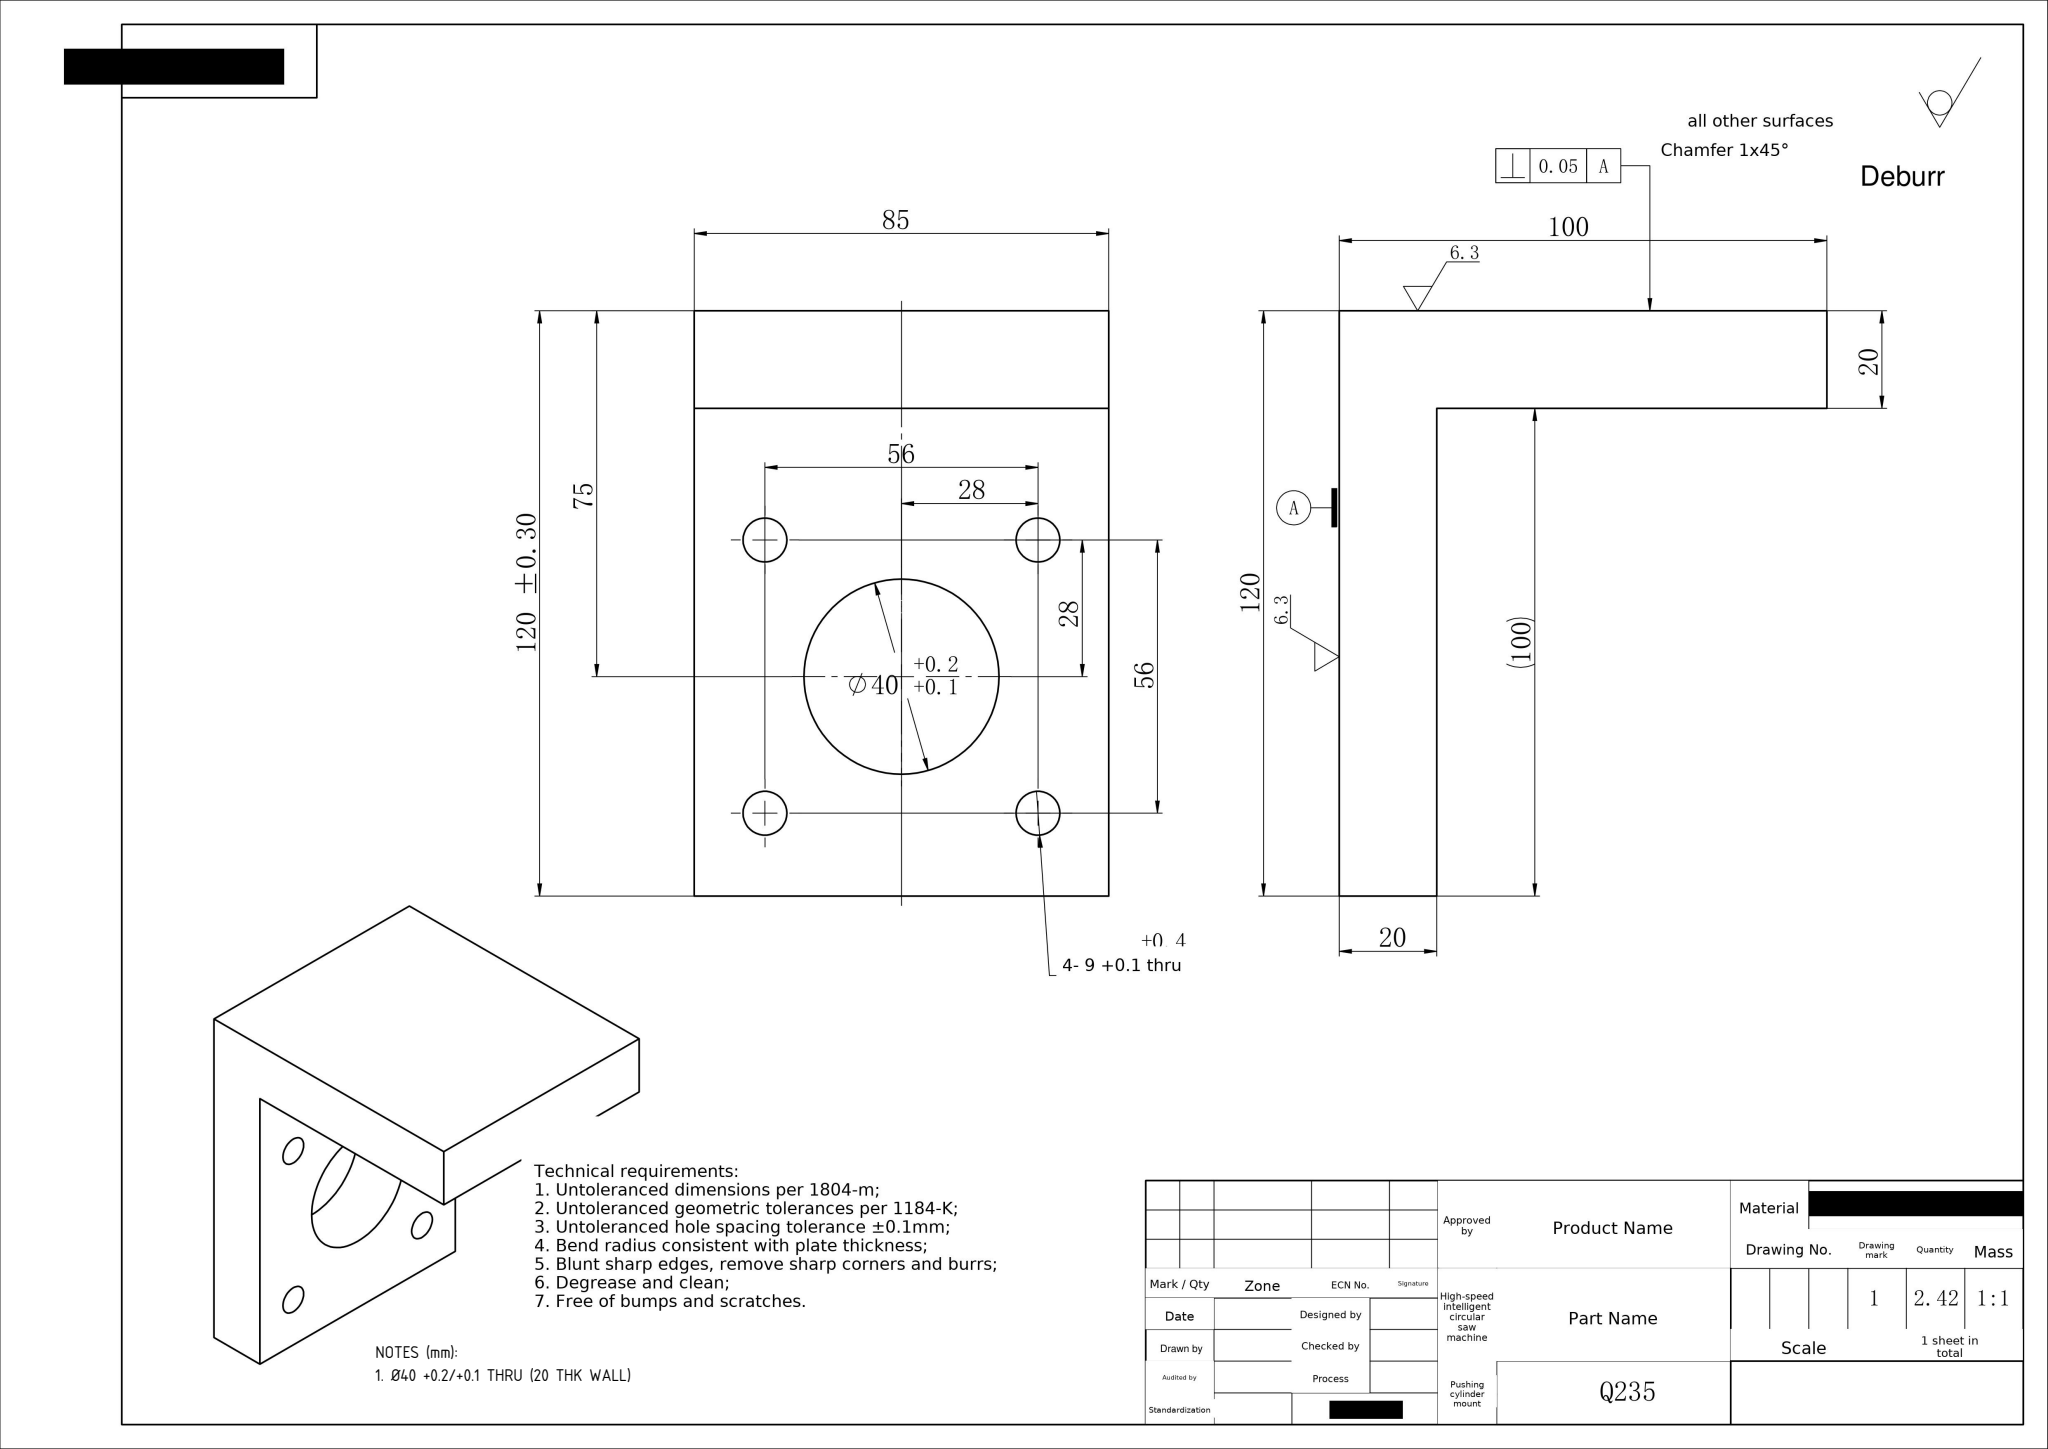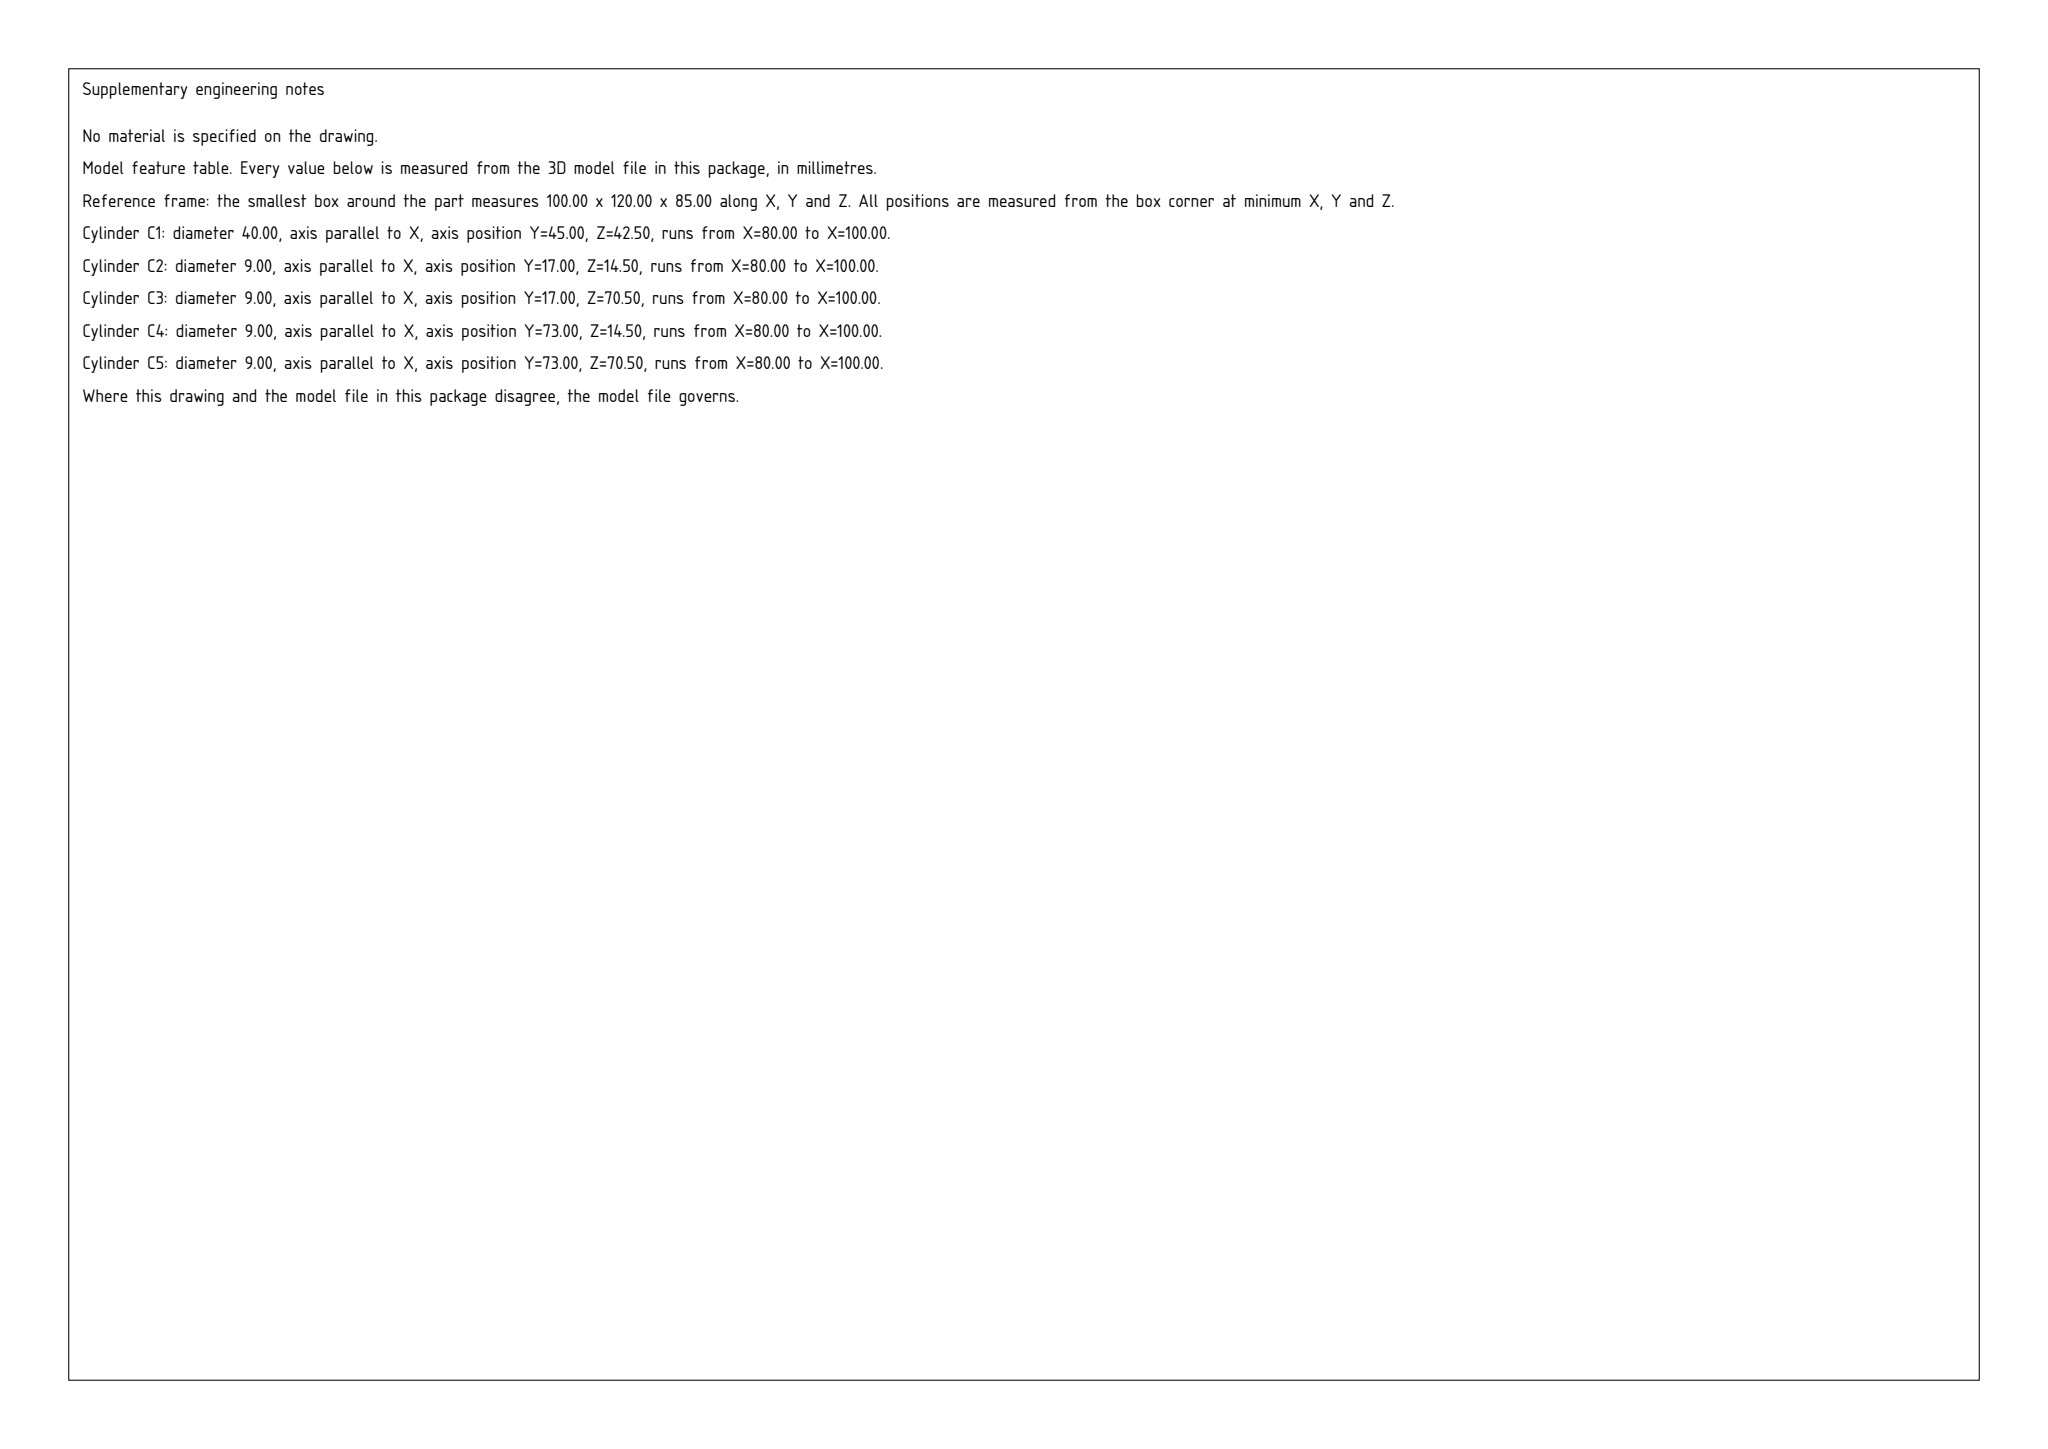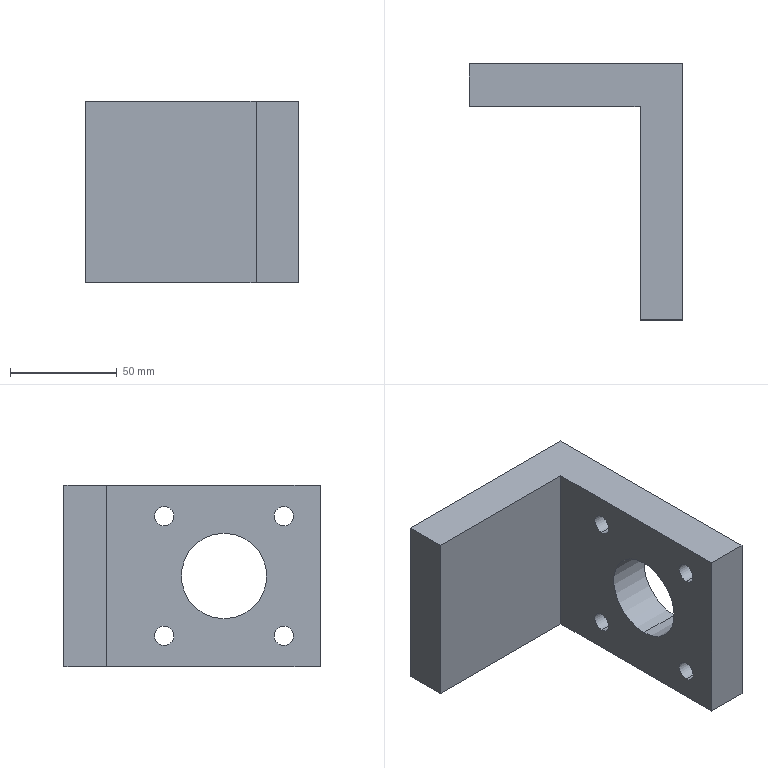Part | SolidWorks | mm | 1 solid | 18 faces | box 100 x 120 x 85 mm | volume 309778 mm3 | cylinder 10 | plane 8 | commonest cylinder face diameters 9 x8 40 x2
Drawing notes:
Ø40 +0.2/+0.1 THRU (20 THK WALL) | from the solid: 40 dia cyl, axis x, length 20.0 = wall thk (x-planes 80.0 to 100.0)
build123d program:
from build123d import *

# Parameters (mm, degrees)
BOSS_EXTRUDE1_DEPTH = 85
SKETCH2_R           = 20
SKETCH2_R_2         = 4.5
CUT_EXTRUDE1_DEPTH  = 178.834


with BuildPart() as part:
    # Sketch1 → Boss-Extrude1 (new body)
    with BuildSketch(Plane.XY):
        Polygon((0, 0), (0, 120), (-100, 120), (-100, 100), (-20, 100), (-20, 0), align=None)
    extrude(amount=BOSS_EXTRUDE1_DEPTH)

    # Sketch2 → Cut-Extrude1 (cut, through all)
    with BuildSketch(Plane(origin=(0, 0, 0), x_dir=(0, 0, -1), z_dir=(1, 0, 0))):
        with Locations((-42.5, 45)):
            Circle(SKETCH2_R)
        with Locations((-70.5, 73)):
            Circle(SKETCH2_R_2)
        with Locations((-14.5, 73)):
            Circle(SKETCH2_R_2)
        with Locations((-14.5, 17)):
            Circle(SKETCH2_R_2)
        with Locations((-70.5, 17)):
            Circle(SKETCH2_R_2)
    extrude(amount=-CUT_EXTRUDE1_DEPTH, mode=Mode.SUBTRACT)


solid = part.part
STEP:
#1=CARTESIAN_POINT('',(-20.,17.,75.));
#2=VERTEX_POINT('',#1);
#3=CARTESIAN_POINT('',(-20.,17.,66.));
#4=VERTEX_POINT('',#3);
#5=CARTESIAN_POINT('',(-20.,17.,70.5));
#6=DIRECTION('',(1.,0.,0.));
#7=DIRECTION('',(0.,0.,-1.));
#8=AXIS2_PLACEMENT_3D('',#5,#6,#7);
#9=CIRCLE('',#8,4.5);
#10=EDGE_CURVE('',#2,#4,#9,.T.);
#11=ORIENTED_EDGE('',*,*,#10,.F.);
#12=CARTESIAN_POINT('',(0.,17.,75.));
#13=VERTEX_POINT('',#12);
#14=CARTESIAN_POINT('',(-100.,17.,75.));
#15=DIRECTION('',(1.,0.,0.));
#16=VECTOR('',#15,1000.);
#17=LINE('',#14,#16);
#18=EDGE_CURVE('',#2,#13,#17,.T.);
#19=ORIENTED_EDGE('',*,*,#18,.T.);
#20=CARTESIAN_POINT('',(0.,17.,66.));
#21=VERTEX_POINT('',#20);
#22=CARTESIAN_POINT('',(0.,17.,70.5));
#23=DIRECTION('',(1.,0.,0.));
#24=DIRECTION('',(0.,0.,1.));
#25=AXIS2_PLACEMENT_3D('',#22,#23,#24);
#26=CIRCLE('',#25,4.5);
#27=EDGE_CURVE('',#13,#21,#26,.T.);
#28=ORIENTED_EDGE('',*,*,#27,.T.);
#29=CARTESIAN_POINT('',(-100.,17.,66.));
#30=DIRECTION('',(1.,0.,0.));
#31=VECTOR('',#30,1000.);
#32=LINE('',#29,#31);
#33=EDGE_CURVE('',#4,#21,#32,.T.);
#34=ORIENTED_EDGE('',*,*,#33,.F.);
#35=EDGE_LOOP('',(#11,#19,#28,#34));
#36=FACE_OUTER_BOUND('',#35,.T.);
#37=CARTESIAN_POINT('',(-100.,17.,70.5));
#38=DIRECTION('',(1.,0.,0.));
#39=DIRECTION('',(0.,0.,-1.));
#40=AXIS2_PLACEMENT_3D('',#37,#38,#39);
#41=CYLINDRICAL_SURFACE('',#40,4.5);
#42=ADVANCED_FACE('',(#36),#41,.F.);
#43=CARTESIAN_POINT('',(-20.,17.,19.));
#44=VERTEX_POINT('',#43);
#45=CARTESIAN_POINT('',(-20.,17.,10.));
#46=VERTEX_POINT('',#45);
#47=CARTESIAN_POINT('',(-20.,17.,14.5));
#48=DIRECTION('',(1.,0.,0.));
#49=DIRECTION('',(0.,0.,-1.));
#50=AXIS2_PLACEMENT_3D('',#47,#48,#49);
#51=CIRCLE('',#50,4.5);
#52=EDGE_CURVE('',#44,#46,#51,.T.);
#53=ORIENTED_EDGE('',*,*,#52,.F.);
#54=CARTESIAN_POINT('',(0.,17.,19.));
#55=VERTEX_POINT('',#54);
#56=CARTESIAN_POINT('',(-100.,17.,19.));
#57=DIRECTION('',(1.,0.,0.));
#58=VECTOR('',#57,1000.);
#59=LINE('',#56,#58);
#60=EDGE_CURVE('',#44,#55,#59,.T.);
#61=ORIENTED_EDGE('',*,*,#60,.T.);
#62=CARTESIAN_POINT('',(0.,17.,10.));
#63=VERTEX_POINT('',#62);
#64=CARTESIAN_POINT('',(0.,17.,14.5));
#65=DIRECTION('',(1.,0.,0.));
#66=DIRECTION('',(0.,0.,-1.));
#67=AXIS2_PLACEMENT_3D('',#64,#65,#66);
#68=CIRCLE('',#67,4.5);
#69=EDGE_CURVE('',#55,#63,#68,.T.);
#70=ORIENTED_EDGE('',*,*,#69,.T.);
#71=CARTESIAN_POINT('',(-100.,17.,10.));
#72=DIRECTION('',(1.,0.,0.));
#73=VECTOR('',#72,1000.);
#74=LINE('',#71,#73);
#75=EDGE_CURVE('',#46,#63,#74,.T.);
#76=ORIENTED_EDGE('',*,*,#75,.F.);
#77=EDGE_LOOP('',(#53,#61,#70,#76));
#78=FACE_OUTER_BOUND('',#77,.T.);
#79=CARTESIAN_POINT('',(-100.,17.,14.5));
#80=DIRECTION('',(1.,0.,0.));
#81=DIRECTION('',(0.,0.,-1.));
#82=AXIS2_PLACEMENT_3D('',#79,#80,#81);
#83=CYLINDRICAL_SURFACE('',#82,4.5);
#84=ADVANCED_FACE('',(#78),#83,.F.);
#85=CARTESIAN_POINT('',(-20.,73.,19.));
#86=VERTEX_POINT('',#85);
#87=CARTESIAN_POINT('',(-20.,73.,10.));
#88=VERTEX_POINT('',#87);
#89=CARTESIAN_POINT('',(-20.,73.,14.5));
#90=DIRECTION('',(1.,0.,0.));
#91=DIRECTION('',(0.,0.,-1.));
#92=AXIS2_PLACEMENT_3D('',#89,#90,#91);
#93=CIRCLE('',#92,4.5);
#94=EDGE_CURVE('',#86,#88,#93,.T.);
#95=ORIENTED_EDGE('',*,*,#94,.F.);
#96=CARTESIAN_POINT('',(0.,73.,19.));
#97=VERTEX_POINT('',#96);
#98=CARTESIAN_POINT('',(-100.,73.,19.));
#99=DIRECTION('',(1.,0.,0.));
#100=VECTOR('',#99,1000.);
#101=LINE('',#98,#100);
#102=EDGE_CURVE('',#86,#97,#101,.T.);
#103=ORIENTED_EDGE('',*,*,#102,.T.);
#104=CARTESIAN_POINT('',(0.,73.,10.));
#105=VERTEX_POINT('',#104);
#106=CARTESIAN_POINT('',(0.,73.,14.5));
#107=DIRECTION('',(1.,0.,0.));
#108=DIRECTION('',(0.,0.,1.));
#109=AXIS2_PLACEMENT_3D('',#106,#107,#108);
#110=CIRCLE('',#109,4.5);
#111=EDGE_CURVE('',#97,#105,#110,.T.);
#112=ORIENTED_EDGE('',*,*,#111,.T.);
#113=CARTESIAN_POINT('',(-100.,73.,10.));
#114=DIRECTION('',(1.,0.,0.));
#115=VECTOR('',#114,1000.);
#116=LINE('',#113,#115);
#117=EDGE_CURVE('',#88,#105,#116,.T.);
#118=ORIENTED_EDGE('',*,*,#117,.F.);
#119=EDGE_LOOP('',(#95,#103,#112,#118));
#120=FACE_OUTER_BOUND('',#119,.T.);
#121=CARTESIAN_POINT('',(-100.,73.,14.5));
#122=DIRECTION('',(1.,0.,0.));
#123=DIRECTION('',(0.,0.,-1.));
#124=AXIS2_PLACEMENT_3D('',#121,#122,#123);
#125=CYLINDRICAL_SURFACE('',#124,4.5);
#126=ADVANCED_FACE('',(#120),#125,.F.);
#127=CARTESIAN_POINT('',(-20.,73.,75.));
#128=VERTEX_POINT('',#127);
#129=CARTESIAN_POINT('',(-20.,73.,66.));
#130=VERTEX_POINT('',#129);
#131=CARTESIAN_POINT('',(-20.,73.,70.5));
#132=DIRECTION('',(1.,0.,0.));
#133=DIRECTION('',(0.,0.,-1.));
#134=AXIS2_PLACEMENT_3D('',#131,#132,#133);
#135=CIRCLE('',#134,4.5);
#136=EDGE_CURVE('',#128,#130,#135,.T.);
#137=ORIENTED_EDGE('',*,*,#136,.F.);
#138=CARTESIAN_POINT('',(0.,73.,75.));
#139=VERTEX_POINT('',#138);
#140=CARTESIAN_POINT('',(-100.,73.,75.));
#141=DIRECTION('',(1.,0.,0.));
#142=VECTOR('',#141,1000.);
#143=LINE('',#140,#142);
#144=EDGE_CURVE('',#128,#139,#143,.T.);
#145=ORIENTED_EDGE('',*,*,#144,.T.);
#146=CARTESIAN_POINT('',(0.,73.,66.));
#147=VERTEX_POINT('',#146);
#148=CARTESIAN_POINT('',(0.,73.,70.5));
#149=DIRECTION('',(1.,0.,0.));
#150=DIRECTION('',(0.,0.,-1.));
#151=AXIS2_PLACEMENT_3D('',#148,#149,#150);
#152=CIRCLE('',#151,4.5);
#153=EDGE_CURVE('',#139,#147,#152,.T.);
#154=ORIENTED_EDGE('',*,*,#153,.T.);
#155=CARTESIAN_POINT('',(-100.,73.,66.));
#156=DIRECTION('',(1.,0.,0.));
#157=VECTOR('',#156,1000.);
#158=LINE('',#155,#157);
#159=EDGE_CURVE('',#130,#147,#158,.T.);
#160=ORIENTED_EDGE('',*,*,#159,.F.);
#161=EDGE_LOOP('',(#137,#145,#154,#160));
#162=FACE_OUTER_BOUND('',#161,.T.);
#163=CARTESIAN_POINT('',(-100.,73.,70.5));
#164=DIRECTION('',(1.,0.,0.));
#165=DIRECTION('',(0.,0.,-1.));
#166=AXIS2_PLACEMENT_3D('',#163,#164,#165);
#167=CYLINDRICAL_SURFACE('',#166,4.5);
#168=ADVANCED_FACE('',(#162),#167,.F.);
#169=CARTESIAN_POINT('',(-20.,45.,62.5));
#170=VERTEX_POINT('',#169);
#171=CARTESIAN_POINT('',(-20.,45.,22.5));
#172=VERTEX_POINT('',#171);
#173=CARTESIAN_POINT('',(-20.,45.,42.5));
#174=DIRECTION('',(1.,0.,0.));
#175=DIRECTION('',(0.,0.,-1.));
#176=AXIS2_PLACEMENT_3D('',#173,#174,#175);
#177=CIRCLE('',#176,20.);
#178=EDGE_CURVE('',#170,#172,#177,.T.);
#179=ORIENTED_EDGE('',*,*,#178,.F.);
#180=CARTESIAN_POINT('',(0.,45.,62.5));
#181=VERTEX_POINT('',#180);
#182=CARTESIAN_POINT('',(-100.,45.,62.5));
#183=DIRECTION('',(1.,0.,0.));
#184=VECTOR('',#183,1000.);
#185=LINE('',#182,#184);
#186=EDGE_CURVE('',#170,#181,#185,.T.);
#187=ORIENTED_EDGE('',*,*,#186,.T.);
#188=CARTESIAN_POINT('',(0.,45.,22.5));
#189=VERTEX_POINT('',#188);
#190=CARTESIAN_POINT('',(0.,45.,42.5));
#191=DIRECTION('',(1.,0.,0.));
#192=DIRECTION('',(0.,0.,-1.));
#193=AXIS2_PLACEMENT_3D('',#190,#191,#192);
#194=CIRCLE('',#193,20.);
#195=EDGE_CURVE('',#181,#189,#194,.T.);
#196=ORIENTED_EDGE('',*,*,#195,.T.);
#197=CARTESIAN_POINT('',(-100.,45.,22.5));
#198=DIRECTION('',(1.,0.,0.));
#199=VECTOR('',#198,1000.);
#200=LINE('',#197,#199);
#201=EDGE_CURVE('',#172,#189,#200,.T.);
#202=ORIENTED_EDGE('',*,*,#201,.F.);
#203=EDGE_LOOP('',(#179,#187,#196,#202));
#204=FACE_OUTER_BOUND('',#203,.T.);
#205=CARTESIAN_POINT('',(-100.,45.,42.5));
#206=DIRECTION('',(1.,0.,0.));
#207=DIRECTION('',(0.,0.,-1.));
#208=AXIS2_PLACEMENT_3D('',#205,#206,#207);
#209=CYLINDRICAL_SURFACE('',#208,20.);
#210=ADVANCED_FACE('',(#204),#209,.F.);
#211=CARTESIAN_POINT('',(-20.,0.,0.));
#212=VERTEX_POINT('',#211);
#213=CARTESIAN_POINT('',(0.,0.,0.));
#214=VERTEX_POINT('',#213);
#215=CARTESIAN_POINT('',(-20.,0.,0.));
#216=DIRECTION('',(1.,0.,0.));
#217=VECTOR('',#216,1000.);
#218=LINE('',#215,#217);
#219=EDGE_CURVE('',#212,#214,#218,.T.);
#220=ORIENTED_EDGE('',*,*,#219,.T.);
#221=CARTESIAN_POINT('',(0.,0.,85.));
#222=VERTEX_POINT('',#221);
#223=CARTESIAN_POINT('',(0.,0.,85.));
#224=DIRECTION('',(0.,0.,-1.));
#225=VECTOR('',#224,1000.);
#226=LINE('',#223,#225);
#227=EDGE_CURVE('',#222,#214,#226,.T.);
#228=ORIENTED_EDGE('',*,*,#227,.F.);
#229=CARTESIAN_POINT('',(-20.,0.,85.));
#230=VERTEX_POINT('',#229);
#231=CARTESIAN_POINT('',(-20.,0.,85.));
#232=DIRECTION('',(1.,0.,0.));
#233=VECTOR('',#232,1000.);
#234=LINE('',#231,#233);
#235=EDGE_CURVE('',#230,#222,#234,.T.);
#236=ORIENTED_EDGE('',*,*,#235,.F.);
#237=CARTESIAN_POINT('',(-20.,0.,85.));
#238=DIRECTION('',(0.,0.,-1.));
#239=VECTOR('',#238,1000.);
#240=LINE('',#237,#239);
#241=EDGE_CURVE('',#230,#212,#240,.T.);
#242=ORIENTED_EDGE('',*,*,#241,.T.);
#243=EDGE_LOOP('',(#220,#228,#236,#242));
#244=FACE_OUTER_BOUND('',#243,.T.);
#245=CARTESIAN_POINT('',(-20.,0.,85.));
#246=DIRECTION('',(0.,1.,0.));
#247=DIRECTION('',(0.,0.,1.));
#248=AXIS2_PLACEMENT_3D('',#245,#246,#247);
#249=PLANE('',#248);
#250=ADVANCED_FACE('',(#244),#249,.F.);
#251=CARTESIAN_POINT('',(0.,17.,70.5));
#252=DIRECTION('',(1.,0.,0.));
#253=DIRECTION('',(0.,0.,1.));
#254=AXIS2_PLACEMENT_3D('',#251,#252,#253);
#255=CIRCLE('',#254,4.5);
#256=EDGE_CURVE('',#21,#13,#255,.T.);
#257=ORIENTED_EDGE('',*,*,#256,.F.);
#258=ORIENTED_EDGE('',*,*,#27,.F.);
#259=EDGE_LOOP('',(#257,#258));
#260=FACE_BOUND('',#259,.T.);
#261=CARTESIAN_POINT('',(0.,17.,14.5));
#262=DIRECTION('',(1.,0.,0.));
#263=DIRECTION('',(0.,0.,-1.));
#264=AXIS2_PLACEMENT_3D('',#261,#262,#263);
#265=CIRCLE('',#264,4.5);
#266=EDGE_CURVE('',#63,#55,#265,.T.);
#267=ORIENTED_EDGE('',*,*,#266,.F.);
#268=ORIENTED_EDGE('',*,*,#69,.F.);
#269=EDGE_LOOP('',(#267,#268));
#270=FACE_BOUND('',#269,.T.);
#271=CARTESIAN_POINT('',(0.,73.,14.5));
#272=DIRECTION('',(1.,0.,0.));
#273=DIRECTION('',(0.,0.,1.));
#274=AXIS2_PLACEMENT_3D('',#271,#272,#273);
#275=CIRCLE('',#274,4.5);
#276=EDGE_CURVE('',#105,#97,#275,.T.);
#277=ORIENTED_EDGE('',*,*,#276,.F.);
#278=ORIENTED_EDGE('',*,*,#111,.F.);
#279=EDGE_LOOP('',(#277,#278));
#280=FACE_BOUND('',#279,.T.);
#281=CARTESIAN_POINT('',(0.,73.,70.5));
#282=DIRECTION('',(1.,0.,0.));
#283=DIRECTION('',(0.,0.,-1.));
#284=AXIS2_PLACEMENT_3D('',#281,#282,#283);
#285=CIRCLE('',#284,4.5);
#286=EDGE_CURVE('',#147,#139,#285,.T.);
#287=ORIENTED_EDGE('',*,*,#286,.F.);
#288=ORIENTED_EDGE('',*,*,#153,.F.);
#289=EDGE_LOOP('',(#287,#288));
#290=FACE_BOUND('',#289,.T.);
#291=CARTESIAN_POINT('',(0.,45.,42.5));
#292=DIRECTION('',(1.,0.,0.));
#293=DIRECTION('',(0.,0.,-1.));
#294=AXIS2_PLACEMENT_3D('',#291,#292,#293);
#295=CIRCLE('',#294,20.);
#296=EDGE_CURVE('',#189,#181,#295,.T.);
#297=ORIENTED_EDGE('',*,*,#296,.F.);
#298=ORIENTED_EDGE('',*,*,#195,.F.);
#299=EDGE_LOOP('',(#297,#298));
#300=FACE_BOUND('',#299,.T.);
#301=CARTESIAN_POINT('',(0.,120.,0.));
#302=VERTEX_POINT('',#301);
#303=CARTESIAN_POINT('',(0.,0.,0.));
#304=DIRECTION('',(0.,1.,0.));
#305=VECTOR('',#304,1000.);
#306=LINE('',#303,#305);
#307=EDGE_CURVE('',#214,#302,#306,.T.);
#308=ORIENTED_EDGE('',*,*,#307,.T.);
#309=CARTESIAN_POINT('',(0.,120.,85.));
#310=VERTEX_POINT('',#309);
#311=CARTESIAN_POINT('',(0.,120.,85.));
#312=DIRECTION('',(0.,0.,-1.));
#313=VECTOR('',#312,1000.);
#314=LINE('',#311,#313);
#315=EDGE_CURVE('',#310,#302,#314,.T.);
#316=ORIENTED_EDGE('',*,*,#315,.F.);
#317=CARTESIAN_POINT('',(0.,0.,85.));
#318=DIRECTION('',(0.,1.,0.));
#319=VECTOR('',#318,1000.);
#320=LINE('',#317,#319);
#321=EDGE_CURVE('',#222,#310,#320,.T.);
#322=ORIENTED_EDGE('',*,*,#321,.F.);
#323=ORIENTED_EDGE('',*,*,#227,.T.);
#324=EDGE_LOOP('',(#308,#316,#322,#323));
#325=FACE_OUTER_BOUND('',#324,.T.);
#326=CARTESIAN_POINT('',(0.,0.,85.));
#327=DIRECTION('',(-1.,0.,0.));
#328=DIRECTION('',(0.,0.,1.));
#329=AXIS2_PLACEMENT_3D('',#326,#327,#328);
#330=PLANE('',#329);
#331=ADVANCED_FACE('',(#260,#270,#280,#290,#300,#325),#330,.F.);
#332=CARTESIAN_POINT('',(-100.,120.,0.));
#333=VERTEX_POINT('',#332);
#334=CARTESIAN_POINT('',(0.,120.,0.));
#335=DIRECTION('',(-1.,-0.,0.));
#336=VECTOR('',#335,1000.);
#337=LINE('',#334,#336);
#338=EDGE_CURVE('',#302,#333,#337,.T.);
#339=ORIENTED_EDGE('',*,*,#338,.T.);
#340=CARTESIAN_POINT('',(-100.,120.,85.));
#341=VERTEX_POINT('',#340);
#342=CARTESIAN_POINT('',(-100.,120.,85.));
#343=DIRECTION('',(0.,0.,-1.));
#344=VECTOR('',#343,1000.);
#345=LINE('',#342,#344);
#346=EDGE_CURVE('',#341,#333,#345,.T.);
#347=ORIENTED_EDGE('',*,*,#346,.F.);
#348=CARTESIAN_POINT('',(0.,120.,85.));
#349=DIRECTION('',(-1.,-0.,0.));
#350=VECTOR('',#349,1000.);
#351=LINE('',#348,#350);
#352=EDGE_CURVE('',#310,#341,#351,.T.);
#353=ORIENTED_EDGE('',*,*,#352,.F.);
#354=ORIENTED_EDGE('',*,*,#315,.T.);
#355=EDGE_LOOP('',(#339,#347,#353,#354));
#356=FACE_OUTER_BOUND('',#355,.T.);
#357=CARTESIAN_POINT('',(0.,120.,85.));
#358=DIRECTION('',(0.,-1.,0.));
#359=DIRECTION('',(1.,0.,0.));
#360=AXIS2_PLACEMENT_3D('',#357,#358,#359);
#361=PLANE('',#360);
#362=ADVANCED_FACE('',(#356),#361,.F.);
#363=CARTESIAN_POINT('',(-100.,100.,0.));
#364=VERTEX_POINT('',#363);
#365=CARTESIAN_POINT('',(-100.,100.,0.));
#366=DIRECTION('',(0.,-1.,0.));
#367=VECTOR('',#366,1000.);
#368=LINE('',#365,#367);
#369=EDGE_CURVE('',#333,#364,#368,.T.);
#370=ORIENTED_EDGE('',*,*,#369,.T.);
#371=CARTESIAN_POINT('',(-100.,100.,85.));
#372=VERTEX_POINT('',#371);
#373=CARTESIAN_POINT('',(-100.,100.,85.));
#374=DIRECTION('',(0.,0.,-1.));
#375=VECTOR('',#374,1000.);
#376=LINE('',#373,#375);
#377=EDGE_CURVE('',#372,#364,#376,.T.);
#378=ORIENTED_EDGE('',*,*,#377,.F.);
#379=CARTESIAN_POINT('',(-100.,100.,85.));
#380=DIRECTION('',(0.,-1.,0.));
#381=VECTOR('',#380,1000.);
#382=LINE('',#379,#381);
#383=EDGE_CURVE('',#341,#372,#382,.T.);
#384=ORIENTED_EDGE('',*,*,#383,.F.);
#385=ORIENTED_EDGE('',*,*,#346,.T.);
#386=EDGE_LOOP('',(#370,#378,#384,#385));
#387=FACE_OUTER_BOUND('',#386,.T.);
#388=CARTESIAN_POINT('',(-100.,100.,85.));
#389=DIRECTION('',(1.,0.,0.));
#390=DIRECTION('',(0.,0.,-1.));
#391=AXIS2_PLACEMENT_3D('',#388,#389,#390);
#392=PLANE('',#391);
#393=ADVANCED_FACE('',(#387),#392,.F.);
#394=CARTESIAN_POINT('',(-20.,100.,0.));
#395=VERTEX_POINT('',#394);
#396=CARTESIAN_POINT('',(-20.,100.,0.));
#397=DIRECTION('',(1.,0.,0.));
#398=VECTOR('',#397,1000.);
#399=LINE('',#396,#398);
#400=EDGE_CURVE('',#364,#395,#399,.T.);
#401=ORIENTED_EDGE('',*,*,#400,.T.);
#402=CARTESIAN_POINT('',(-20.,100.,85.));
#403=VERTEX_POINT('',#402);
#404=CARTESIAN_POINT('',(-20.,100.,85.));
#405=DIRECTION('',(0.,0.,-1.));
#406=VECTOR('',#405,1000.);
#407=LINE('',#404,#406);
#408=EDGE_CURVE('',#403,#395,#407,.T.);
#409=ORIENTED_EDGE('',*,*,#408,.F.);
#410=CARTESIAN_POINT('',(-20.,100.,85.));
#411=DIRECTION('',(1.,0.,0.));
#412=VECTOR('',#411,1000.);
#413=LINE('',#410,#412);
#414=EDGE_CURVE('',#372,#403,#413,.T.);
#415=ORIENTED_EDGE('',*,*,#414,.F.);
#416=ORIENTED_EDGE('',*,*,#377,.T.);
#417=EDGE_LOOP('',(#401,#409,#415,#416));
#418=FACE_OUTER_BOUND('',#417,.T.);
#419=CARTESIAN_POINT('',(-20.,100.,85.));
#420=DIRECTION('',(-0.,1.,0.));
#421=DIRECTION('',(-1.,-0.,0.));
#422=AXIS2_PLACEMENT_3D('',#419,#420,#421);
#423=PLANE('',#422);
#424=ADVANCED_FACE('',(#418),#423,.F.);
#425=CARTESIAN_POINT('',(-20.,17.,70.5));
#426=DIRECTION('',(1.,0.,0.));
#427=DIRECTION('',(0.,0.,-1.));
#428=AXIS2_PLACEMENT_3D('',#425,#426,#427);
#429=CIRCLE('',#428,4.5);
#430=EDGE_CURVE('',#4,#2,#429,.T.);
#431=ORIENTED_EDGE('',*,*,#430,.T.);
#432=ORIENTED_EDGE('',*,*,#10,.T.);
#433=EDGE_LOOP('',(#431,#432));
#434=FACE_BOUND('',#433,.T.);
#435=CARTESIAN_POINT('',(-20.,17.,14.5));
#436=DIRECTION('',(1.,0.,0.));
#437=DIRECTION('',(0.,0.,-1.));
#438=AXIS2_PLACEMENT_3D('',#435,#436,#437);
#439=CIRCLE('',#438,4.5);
#440=EDGE_CURVE('',#46,#44,#439,.T.);
#441=ORIENTED_EDGE('',*,*,#440,.T.);
#442=ORIENTED_EDGE('',*,*,#52,.T.);
#443=EDGE_LOOP('',(#441,#442));
#444=FACE_BOUND('',#443,.T.);
#445=CARTESIAN_POINT('',(-20.,73.,14.5));
#446=DIRECTION('',(1.,0.,0.));
#447=DIRECTION('',(0.,0.,-1.));
#448=AXIS2_PLACEMENT_3D('',#445,#446,#447);
#449=CIRCLE('',#448,4.5);
#450=EDGE_CURVE('',#88,#86,#449,.T.);
#451=ORIENTED_EDGE('',*,*,#450,.T.);
#452=ORIENTED_EDGE('',*,*,#94,.T.);
#453=EDGE_LOOP('',(#451,#452));
#454=FACE_BOUND('',#453,.T.);
#455=CARTESIAN_POINT('',(-20.,73.,70.5));
#456=DIRECTION('',(1.,0.,0.));
#457=DIRECTION('',(0.,0.,-1.));
#458=AXIS2_PLACEMENT_3D('',#455,#456,#457);
#459=CIRCLE('',#458,4.5);
#460=EDGE_CURVE('',#130,#128,#459,.T.);
#461=ORIENTED_EDGE('',*,*,#460,.T.);
#462=ORIENTED_EDGE('',*,*,#136,.T.);
#463=EDGE_LOOP('',(#461,#462));
#464=FACE_BOUND('',#463,.T.);
#465=CARTESIAN_POINT('',(-20.,45.,42.5));
#466=DIRECTION('',(1.,0.,0.));
#467=DIRECTION('',(0.,0.,-1.));
#468=AXIS2_PLACEMENT_3D('',#465,#466,#467);
#469=CIRCLE('',#468,20.);
#470=EDGE_CURVE('',#172,#170,#469,.T.);
#471=ORIENTED_EDGE('',*,*,#470,.T.);
#472=ORIENTED_EDGE('',*,*,#178,.T.);
#473=EDGE_LOOP('',(#471,#472));
#474=FACE_BOUND('',#473,.T.);
#475=CARTESIAN_POINT('',(-20.,0.,0.));
#476=DIRECTION('',(0.,-1.,0.));
#477=VECTOR('',#476,1000.);
#478=LINE('',#475,#477);
#479=EDGE_CURVE('',#395,#212,#478,.T.);
#480=ORIENTED_EDGE('',*,*,#479,.T.);
#481=ORIENTED_EDGE('',*,*,#241,.F.);
#482=CARTESIAN_POINT('',(-20.,0.,85.));
#483=DIRECTION('',(0.,-1.,0.));
#484=VECTOR('',#483,1000.);
#485=LINE('',#482,#484);
#486=EDGE_CURVE('',#403,#230,#485,.T.);
#487=ORIENTED_EDGE('',*,*,#486,.F.);
#488=ORIENTED_EDGE('',*,*,#408,.T.);
#489=EDGE_LOOP('',(#480,#481,#487,#488));
#490=FACE_OUTER_BOUND('',#489,.T.);
#491=CARTESIAN_POINT('',(-20.,0.,85.));
#492=DIRECTION('',(1.,0.,0.));
#493=DIRECTION('',(0.,0.,-1.));
#494=AXIS2_PLACEMENT_3D('',#491,#492,#493);
#495=PLANE('',#494);
#496=ADVANCED_FACE('',(#434,#444,#454,#464,#474,#490),#495,.F.);
#497=ORIENTED_EDGE('',*,*,#235,.T.);
#498=ORIENTED_EDGE('',*,*,#321,.T.);
#499=ORIENTED_EDGE('',*,*,#352,.T.);
#500=ORIENTED_EDGE('',*,*,#383,.T.);
#501=ORIENTED_EDGE('',*,*,#414,.T.);
#502=ORIENTED_EDGE('',*,*,#486,.T.);
#503=EDGE_LOOP('',(#497,#498,#499,#500,#501,#502));
#504=FACE_OUTER_BOUND('',#503,.T.);
#505=CARTESIAN_POINT('',(0.,0.,85.));
#506=DIRECTION('',(0.,0.,1.));
#507=DIRECTION('',(1.,0.,0.));
#508=AXIS2_PLACEMENT_3D('',#505,#506,#507);
#509=PLANE('',#508);
#510=ADVANCED_FACE('',(#504),#509,.T.);
#511=ORIENTED_EDGE('',*,*,#219,.F.);
#512=ORIENTED_EDGE('',*,*,#479,.F.);
#513=ORIENTED_EDGE('',*,*,#400,.F.);
#514=ORIENTED_EDGE('',*,*,#369,.F.);
#515=ORIENTED_EDGE('',*,*,#338,.F.);
#516=ORIENTED_EDGE('',*,*,#307,.F.);
#517=EDGE_LOOP('',(#511,#512,#513,#514,#515,#516));
#518=FACE_OUTER_BOUND('',#517,.T.);
#519=CARTESIAN_POINT('',(0.,0.,0.));
#520=DIRECTION('',(0.,0.,1.));
#521=DIRECTION('',(1.,0.,0.));
#522=AXIS2_PLACEMENT_3D('',#519,#520,#521);
#523=PLANE('',#522);
#524=ADVANCED_FACE('',(#518),#523,.F.);
#525=ORIENTED_EDGE('',*,*,#186,.F.);
#526=ORIENTED_EDGE('',*,*,#470,.F.);
#527=ORIENTED_EDGE('',*,*,#201,.T.);
#528=ORIENTED_EDGE('',*,*,#296,.T.);
#529=EDGE_LOOP('',(#525,#526,#527,#528));
#530=FACE_OUTER_BOUND('',#529,.T.);
#531=CARTESIAN_POINT('',(-100.,45.,42.5));
#532=DIRECTION('',(1.,0.,0.));
#533=DIRECTION('',(0.,0.,-1.));
#534=AXIS2_PLACEMENT_3D('',#531,#532,#533);
#535=CYLINDRICAL_SURFACE('',#534,20.);
#536=ADVANCED_FACE('',(#530),#535,.F.);
#537=ORIENTED_EDGE('',*,*,#144,.F.);
#538=ORIENTED_EDGE('',*,*,#460,.F.);
#539=ORIENTED_EDGE('',*,*,#159,.T.);
#540=ORIENTED_EDGE('',*,*,#286,.T.);
#541=EDGE_LOOP('',(#537,#538,#539,#540));
#542=FACE_OUTER_BOUND('',#541,.T.);
#543=CARTESIAN_POINT('',(-100.,73.,70.5));
#544=DIRECTION('',(1.,0.,0.));
#545=DIRECTION('',(0.,0.,-1.));
#546=AXIS2_PLACEMENT_3D('',#543,#544,#545);
#547=CYLINDRICAL_SURFACE('',#546,4.5);
#548=ADVANCED_FACE('',(#542),#547,.F.);
#549=ORIENTED_EDGE('',*,*,#102,.F.);
#550=ORIENTED_EDGE('',*,*,#450,.F.);
#551=ORIENTED_EDGE('',*,*,#117,.T.);
#552=ORIENTED_EDGE('',*,*,#276,.T.);
#553=EDGE_LOOP('',(#549,#550,#551,#552));
#554=FACE_OUTER_BOUND('',#553,.T.);
#555=CARTESIAN_POINT('',(-100.,73.,14.5));
#556=DIRECTION('',(1.,0.,0.));
#557=DIRECTION('',(0.,0.,-1.));
#558=AXIS2_PLACEMENT_3D('',#555,#556,#557);
#559=CYLINDRICAL_SURFACE('',#558,4.5);
#560=ADVANCED_FACE('',(#554),#559,.F.);
#561=ORIENTED_EDGE('',*,*,#60,.F.);
#562=ORIENTED_EDGE('',*,*,#440,.F.);
#563=ORIENTED_EDGE('',*,*,#75,.T.);
#564=ORIENTED_EDGE('',*,*,#266,.T.);
#565=EDGE_LOOP('',(#561,#562,#563,#564));
#566=FACE_OUTER_BOUND('',#565,.T.);
#567=CARTESIAN_POINT('',(-100.,17.,14.5));
#568=DIRECTION('',(1.,0.,0.));
#569=DIRECTION('',(0.,0.,-1.));
#570=AXIS2_PLACEMENT_3D('',#567,#568,#569);
#571=CYLINDRICAL_SURFACE('',#570,4.5);
#572=ADVANCED_FACE('',(#566),#571,.F.);
#573=ORIENTED_EDGE('',*,*,#18,.F.);
#574=ORIENTED_EDGE('',*,*,#430,.F.);
#575=ORIENTED_EDGE('',*,*,#33,.T.);
#576=ORIENTED_EDGE('',*,*,#256,.T.);
#577=EDGE_LOOP('',(#573,#574,#575,#576));
#578=FACE_OUTER_BOUND('',#577,.T.);
#579=CARTESIAN_POINT('',(-100.,17.,70.5));
#580=DIRECTION('',(1.,0.,0.));
#581=DIRECTION('',(0.,0.,-1.));
#582=AXIS2_PLACEMENT_3D('',#579,#580,#581);
#583=CYLINDRICAL_SURFACE('',#582,4.5);
#584=ADVANCED_FACE('',(#578),#583,.F.);
#585=CLOSED_SHELL('',(#42,#84,#126,#168,#210,#250,#331,#362,#393,#424,#496,#510,#524,#536,#548,#560,#572,#584));
#586=MANIFOLD_SOLID_BREP('',#585);
#587=CARTESIAN_POINT('',(0.,0.,0.));
#588=DIRECTION('',(0.,0.,1.));
#589=DIRECTION('',(1.,0.,0.));
#590=AXIS2_PLACEMENT_3D('',#587,#588,#589);
#591=(LENGTH_UNIT()NAMED_UNIT(*)SI_UNIT(.MILLI.,.METRE.));
#592=UNCERTAINTY_MEASURE_WITH_UNIT(LENGTH_MEASURE(0.00001),#591,'','');
#593=(NAMED_UNIT(*)PLANE_ANGLE_UNIT()SI_UNIT($,.RADIAN.));
#594=(NAMED_UNIT(*)SI_UNIT($,.STERADIAN.)SOLID_ANGLE_UNIT());
#595=(GEOMETRIC_REPRESENTATION_CONTEXT(3)GLOBAL_UNCERTAINTY_ASSIGNED_CONTEXT((#592))GLOBAL_UNIT_ASSIGNED_CONTEXT((#591,#593,#594))REPRESENTATION_CONTEXT('',''));
#596=ADVANCED_BREP_SHAPE_REPRESENTATION('',(#586,#590),#595);